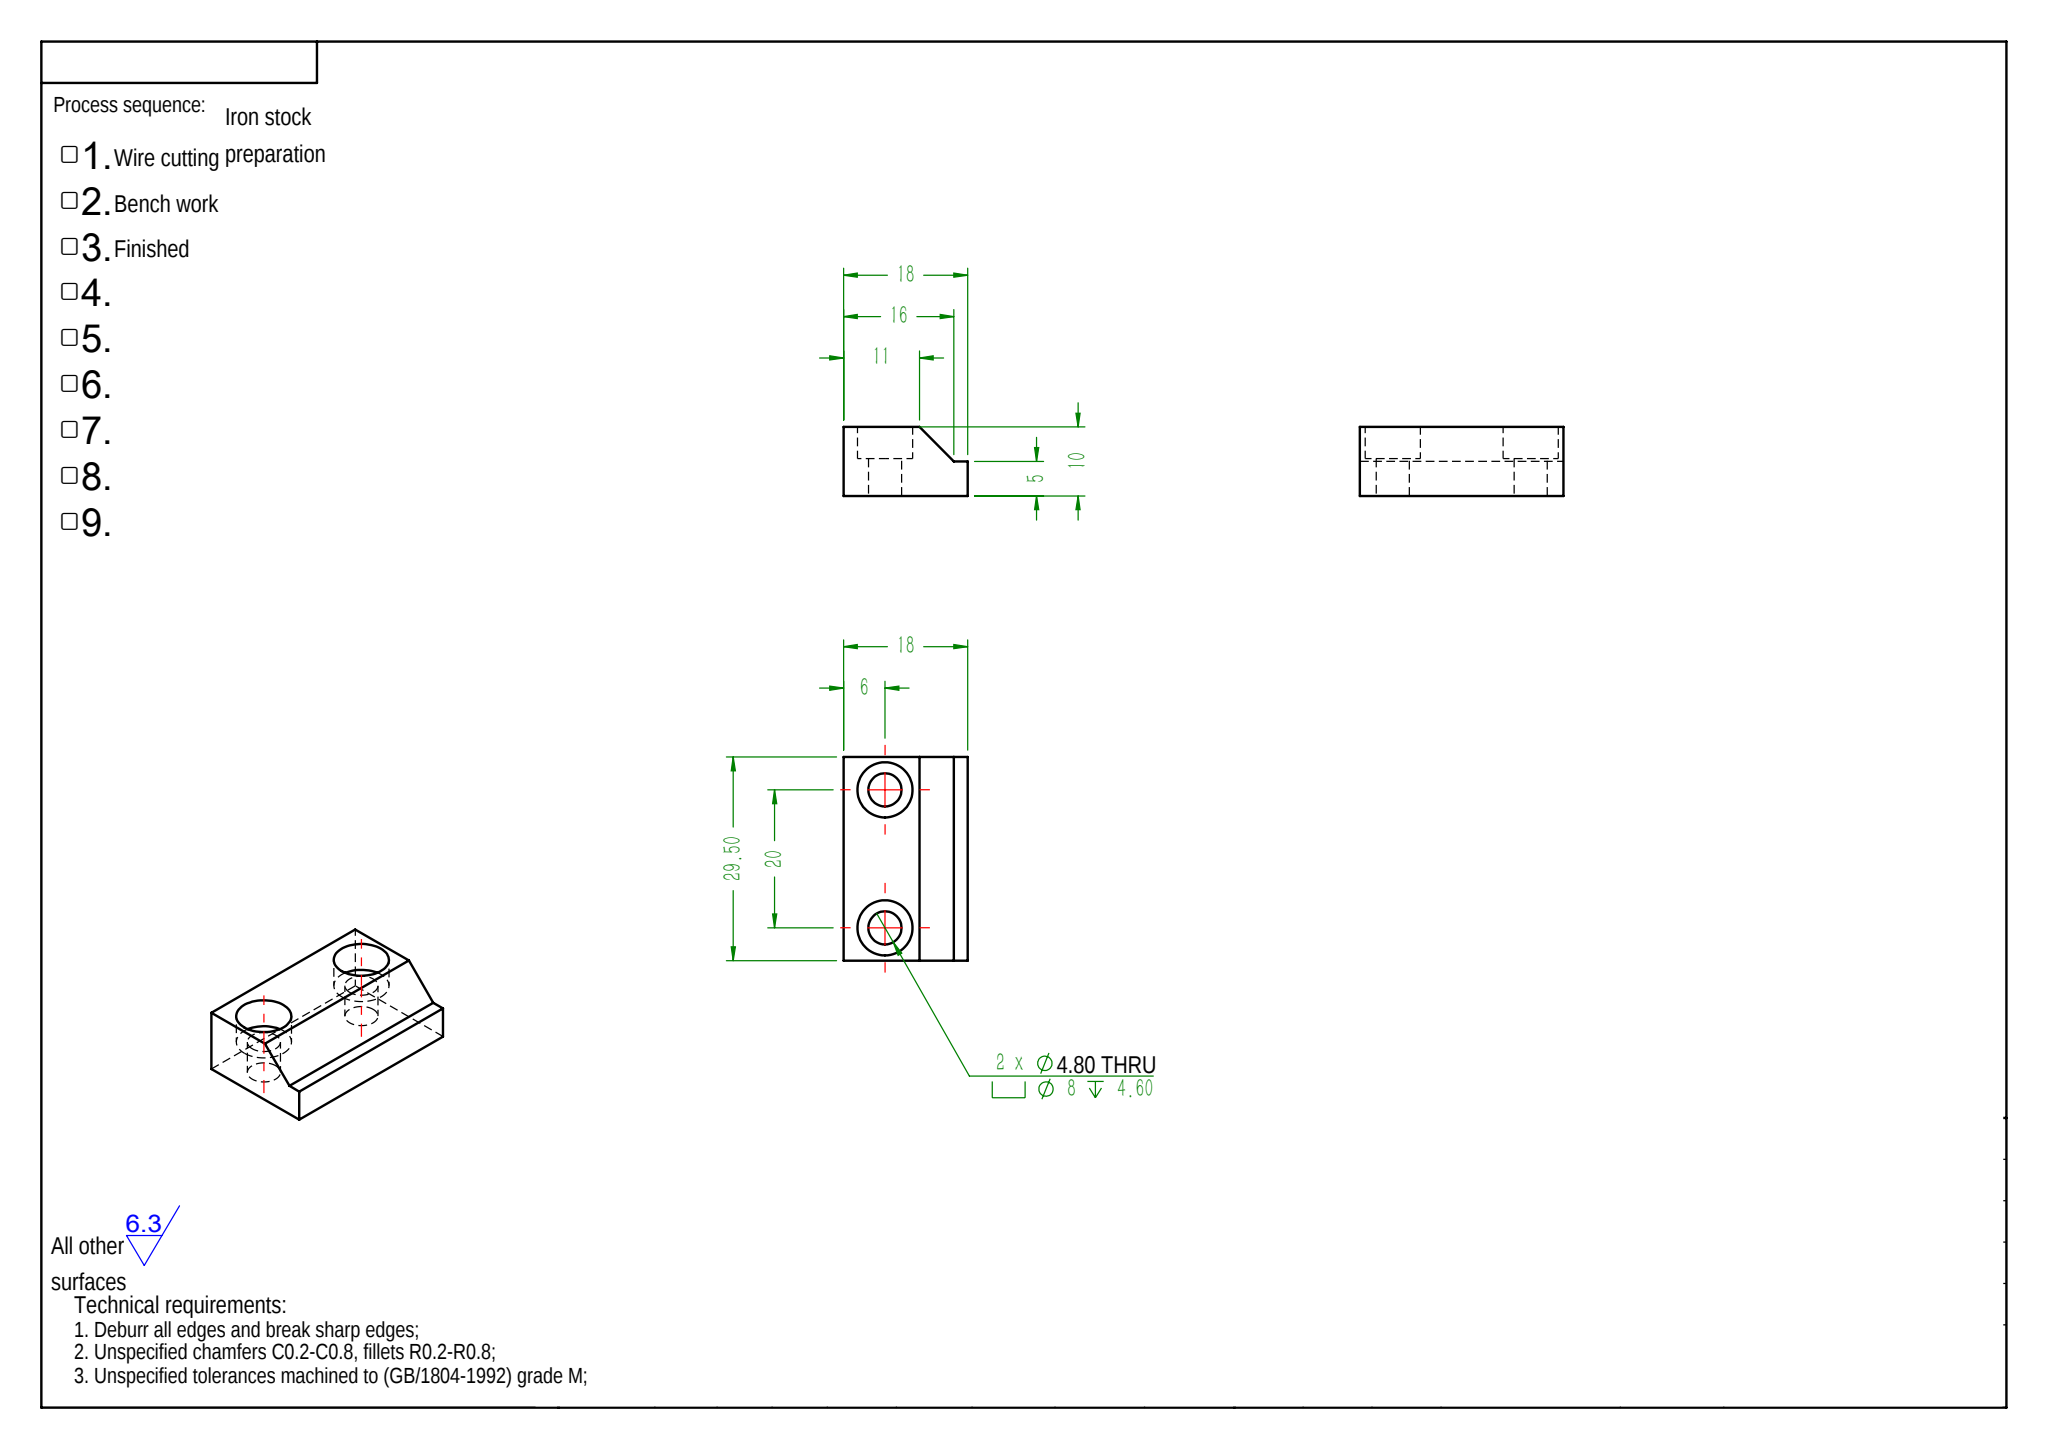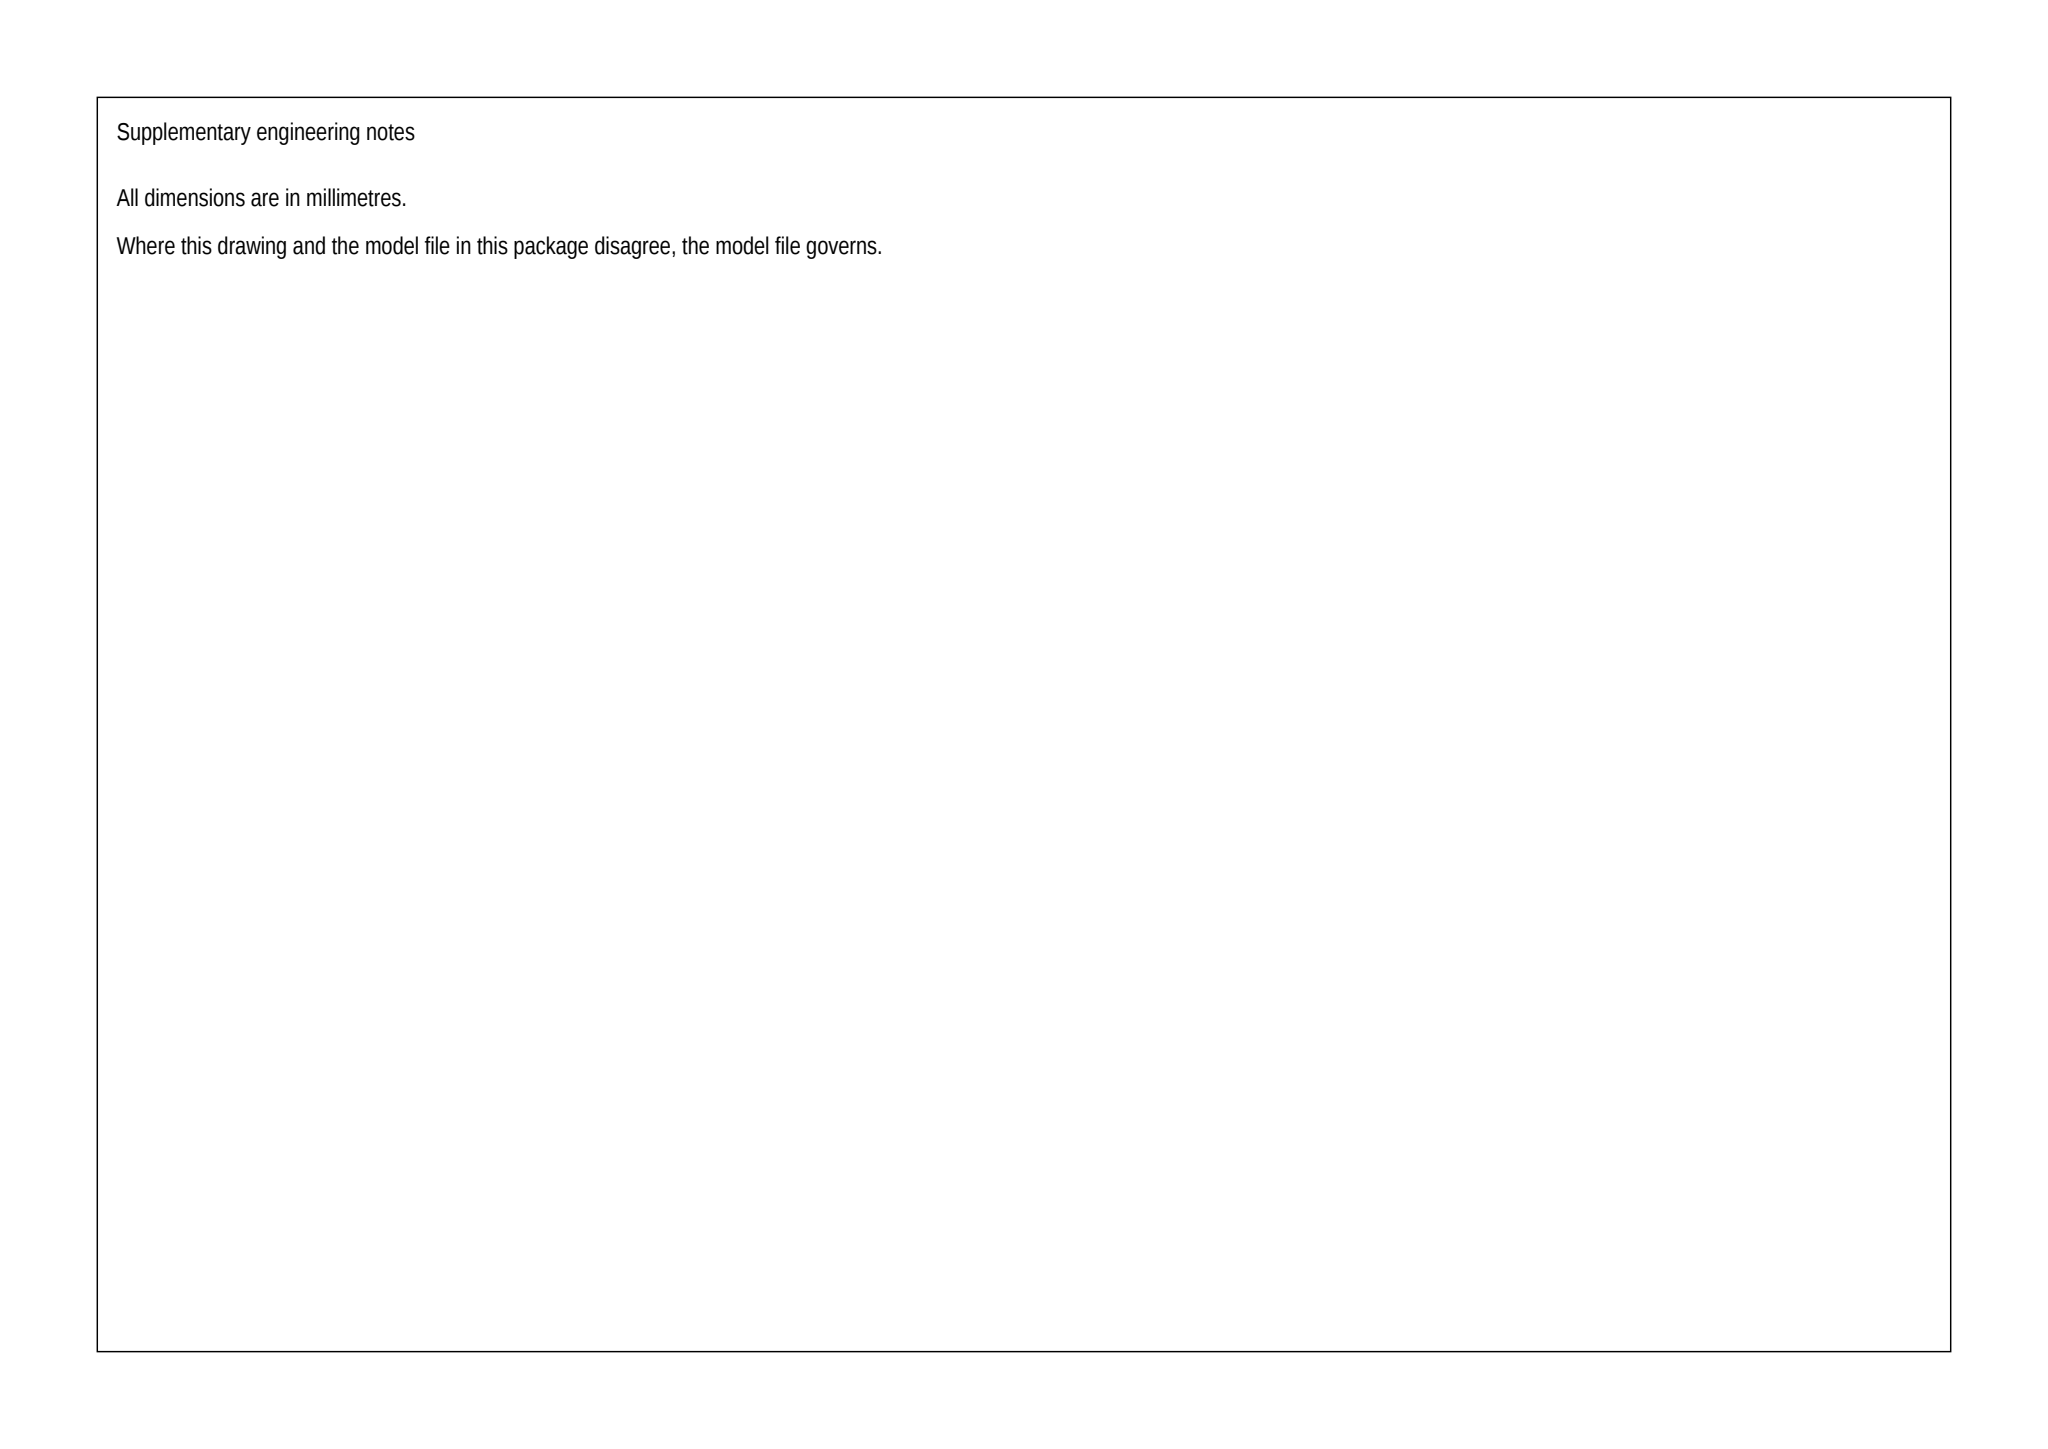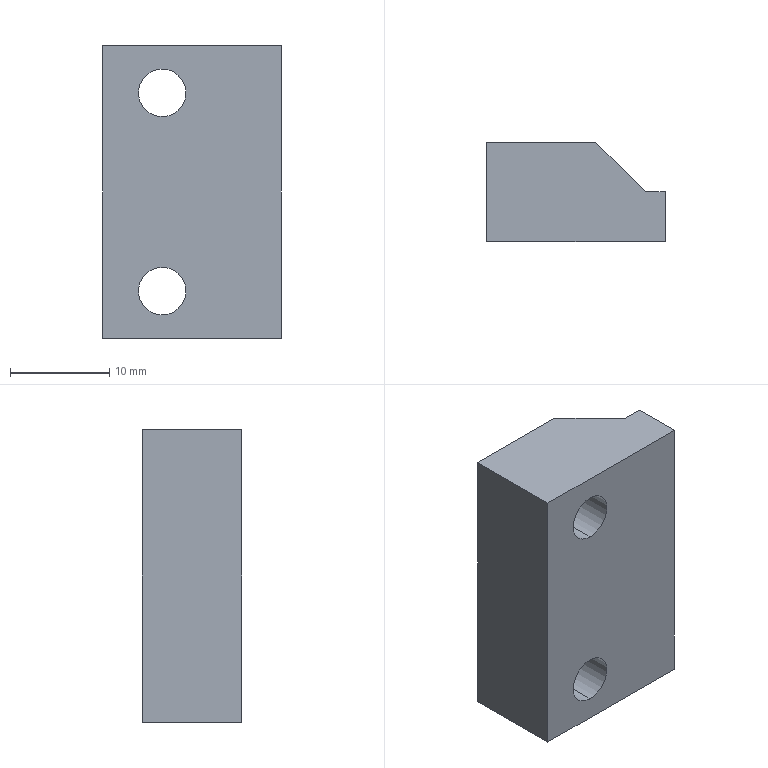Part | SolidWorks | mm | 1 solid | 18 faces | box 18 x 10 x 29.5 mm | volume 3988 mm3 | plane 10 | cylinder 8 | commonest cylinder face diameters 8 x4 4.8 x4
build123d program:
from build123d import *

# Parameters (mm, degrees)
SKETCH2_W                                         = 18
SKETCH2_H                                         = 29.5
BOSS_EXTRUDE1_DEPTH                               = 10
CUT_EXTRUDE1_DEPTH                                = 33.423
HOLE_SIZE_ACCORDING_TO_TYPE_1_OF_HEXA_D           = 4.8
HOLE_SIZE_ACCORDING_TO_TYPE_1_OF_HEXA_CBORE_D     = 8
HOLE_SIZE_ACCORDING_TO_TYPE_1_OF_HEXA_CBORE_DEPTH = 4.6


with BuildPart() as part:
    # Sketch2 → Boss-Extrude1 (new body)
    with BuildSketch(Plane(origin=(0, 0, 0), x_dir=(1, 0, 0), z_dir=(0, 1, 0))):
        Rectangle(SKETCH2_W, SKETCH2_H)
    extrude(amount=BOSS_EXTRUDE1_DEPTH)

    # Sketch3 → Cut-Extrude1 (cut, through all)
    with BuildSketch(Plane.XY.offset(14.75)):
        Polygon((9, 5), (7, 5), (2, 10), (9, 10), align=None)
    extrude(amount=-CUT_EXTRUDE1_DEPTH, mode=Mode.SUBTRACT)

    # Hole Size _ according to_ Type 1 of Hexa (through all)
    with Locations(Plane(origin=(0, 10, 0), x_dir=(1, 0, 0), z_dir=(0, 1, 0))):
        with Locations((-3, 10), (-3, -10)):
            CounterBoreHole(HOLE_SIZE_ACCORDING_TO_TYPE_1_OF_HEXA_D / 2, HOLE_SIZE_ACCORDING_TO_TYPE_1_OF_HEXA_CBORE_D / 2, HOLE_SIZE_ACCORDING_TO_TYPE_1_OF_HEXA_CBORE_DEPTH)


solid = part.part
STEP:
#1=CARTESIAN_POINT('',(-3.,5.4,-14.));
#2=VERTEX_POINT('',#1);
#3=CARTESIAN_POINT('',(-3.,5.4,-6.));
#4=VERTEX_POINT('',#3);
#5=CARTESIAN_POINT('',(-3.,5.4,-10.));
#6=DIRECTION('',(0.,1.,0.));
#7=DIRECTION('',(0.,0.,1.));
#8=AXIS2_PLACEMENT_3D('',#5,#6,#7);
#9=CIRCLE('',#8,4.);
#10=EDGE_CURVE('',#2,#4,#9,.T.);
#11=ORIENTED_EDGE('',*,*,#10,.F.);
#12=CARTESIAN_POINT('',(-3.,10.,-14.));
#13=VERTEX_POINT('',#12);
#14=CARTESIAN_POINT('',(-3.,10.,-14.));
#15=DIRECTION('',(0.,1.,0.));
#16=VECTOR('',#15,1000.);
#17=LINE('',#14,#16);
#18=EDGE_CURVE('',#2,#13,#17,.T.);
#19=ORIENTED_EDGE('',*,*,#18,.T.);
#20=CARTESIAN_POINT('',(-3.,10.,-6.));
#21=VERTEX_POINT('',#20);
#22=CARTESIAN_POINT('',(-3.,10.,-10.));
#23=DIRECTION('',(0.,1.,0.));
#24=DIRECTION('',(0.,0.,1.));
#25=AXIS2_PLACEMENT_3D('',#22,#23,#24);
#26=CIRCLE('',#25,4.);
#27=EDGE_CURVE('',#13,#21,#26,.T.);
#28=ORIENTED_EDGE('',*,*,#27,.T.);
#29=CARTESIAN_POINT('',(-3.,10.,-6.));
#30=DIRECTION('',(0.,1.,0.));
#31=VECTOR('',#30,1000.);
#32=LINE('',#29,#31);
#33=EDGE_CURVE('',#4,#21,#32,.T.);
#34=ORIENTED_EDGE('',*,*,#33,.F.);
#35=EDGE_LOOP('',(#11,#19,#28,#34));
#36=FACE_OUTER_BOUND('',#35,.T.);
#37=CARTESIAN_POINT('',(-3.,10.,-10.));
#38=DIRECTION('',(0.,1.,0.));
#39=DIRECTION('',(0.,0.,1.));
#40=AXIS2_PLACEMENT_3D('',#37,#38,#39);
#41=CYLINDRICAL_SURFACE('',#40,4.);
#42=ADVANCED_FACE('',(#36),#41,.F.);
#43=CARTESIAN_POINT('',(-3.,0.,-7.6));
#44=VERTEX_POINT('',#43);
#45=CARTESIAN_POINT('',(-3.,0.,-12.4));
#46=VERTEX_POINT('',#45);
#47=CARTESIAN_POINT('',(-3.,0.,-10.));
#48=DIRECTION('',(0.,-1.,0.));
#49=DIRECTION('',(0.,0.,-1.));
#50=AXIS2_PLACEMENT_3D('',#47,#48,#49);
#51=CIRCLE('',#50,2.4);
#52=EDGE_CURVE('',#44,#46,#51,.T.);
#53=ORIENTED_EDGE('',*,*,#52,.T.);
#54=CARTESIAN_POINT('',(-3.,5.4,-12.4));
#55=VERTEX_POINT('',#54);
#56=CARTESIAN_POINT('',(-3.,10.,-12.4));
#57=DIRECTION('',(0.,1.,0.));
#58=VECTOR('',#57,1000.);
#59=LINE('',#56,#58);
#60=EDGE_CURVE('',#46,#55,#59,.T.);
#61=ORIENTED_EDGE('',*,*,#60,.T.);
#62=CARTESIAN_POINT('',(-3.,5.4,-7.6));
#63=VERTEX_POINT('',#62);
#64=CARTESIAN_POINT('',(-3.,5.4,-10.));
#65=DIRECTION('',(0.,1.,0.));
#66=DIRECTION('',(0.,0.,1.));
#67=AXIS2_PLACEMENT_3D('',#64,#65,#66);
#68=CIRCLE('',#67,2.4);
#69=EDGE_CURVE('',#55,#63,#68,.T.);
#70=ORIENTED_EDGE('',*,*,#69,.T.);
#71=CARTESIAN_POINT('',(-3.,10.,-7.6));
#72=DIRECTION('',(0.,1.,0.));
#73=VECTOR('',#72,1000.);
#74=LINE('',#71,#73);
#75=EDGE_CURVE('',#44,#63,#74,.T.);
#76=ORIENTED_EDGE('',*,*,#75,.F.);
#77=EDGE_LOOP('',(#53,#61,#70,#76));
#78=FACE_OUTER_BOUND('',#77,.T.);
#79=CARTESIAN_POINT('',(-3.,10.,-10.));
#80=DIRECTION('',(0.,1.,0.));
#81=DIRECTION('',(0.,0.,1.));
#82=AXIS2_PLACEMENT_3D('',#79,#80,#81);
#83=CYLINDRICAL_SURFACE('',#82,2.4);
#84=ADVANCED_FACE('',(#78),#83,.F.);
#85=CARTESIAN_POINT('',(-3.,5.4,6.));
#86=VERTEX_POINT('',#85);
#87=CARTESIAN_POINT('',(-3.,5.4,14.));
#88=VERTEX_POINT('',#87);
#89=CARTESIAN_POINT('',(-3.,5.4,10.));
#90=DIRECTION('',(0.,1.,0.));
#91=DIRECTION('',(0.,0.,1.));
#92=AXIS2_PLACEMENT_3D('',#89,#90,#91);
#93=CIRCLE('',#92,4.);
#94=EDGE_CURVE('',#86,#88,#93,.T.);
#95=ORIENTED_EDGE('',*,*,#94,.F.);
#96=CARTESIAN_POINT('',(-3.,10.,6.));
#97=VERTEX_POINT('',#96);
#98=CARTESIAN_POINT('',(-3.,10.,6.));
#99=DIRECTION('',(0.,1.,0.));
#100=VECTOR('',#99,1000.);
#101=LINE('',#98,#100);
#102=EDGE_CURVE('',#86,#97,#101,.T.);
#103=ORIENTED_EDGE('',*,*,#102,.T.);
#104=CARTESIAN_POINT('',(-3.,10.,14.));
#105=VERTEX_POINT('',#104);
#106=CARTESIAN_POINT('',(-3.,10.,10.));
#107=DIRECTION('',(0.,1.,0.));
#108=DIRECTION('',(0.,0.,1.));
#109=AXIS2_PLACEMENT_3D('',#106,#107,#108);
#110=CIRCLE('',#109,4.);
#111=EDGE_CURVE('',#97,#105,#110,.T.);
#112=ORIENTED_EDGE('',*,*,#111,.T.);
#113=CARTESIAN_POINT('',(-3.,10.,14.));
#114=DIRECTION('',(0.,1.,0.));
#115=VECTOR('',#114,1000.);
#116=LINE('',#113,#115);
#117=EDGE_CURVE('',#88,#105,#116,.T.);
#118=ORIENTED_EDGE('',*,*,#117,.F.);
#119=EDGE_LOOP('',(#95,#103,#112,#118));
#120=FACE_OUTER_BOUND('',#119,.T.);
#121=CARTESIAN_POINT('',(-3.,10.,10.));
#122=DIRECTION('',(0.,1.,0.));
#123=DIRECTION('',(0.,0.,1.));
#124=AXIS2_PLACEMENT_3D('',#121,#122,#123);
#125=CYLINDRICAL_SURFACE('',#124,4.);
#126=ADVANCED_FACE('',(#120),#125,.F.);
#127=CARTESIAN_POINT('',(-3.,0.,12.4));
#128=VERTEX_POINT('',#127);
#129=CARTESIAN_POINT('',(-3.,0.,7.6));
#130=VERTEX_POINT('',#129);
#131=CARTESIAN_POINT('',(-3.,0.,10.));
#132=DIRECTION('',(0.,-1.,0.));
#133=DIRECTION('',(0.,0.,-1.));
#134=AXIS2_PLACEMENT_3D('',#131,#132,#133);
#135=CIRCLE('',#134,2.4);
#136=EDGE_CURVE('',#128,#130,#135,.T.);
#137=ORIENTED_EDGE('',*,*,#136,.T.);
#138=CARTESIAN_POINT('',(-3.,5.4,7.6));
#139=VERTEX_POINT('',#138);
#140=CARTESIAN_POINT('',(-3.,10.,7.6));
#141=DIRECTION('',(0.,1.,0.));
#142=VECTOR('',#141,1000.);
#143=LINE('',#140,#142);
#144=EDGE_CURVE('',#130,#139,#143,.T.);
#145=ORIENTED_EDGE('',*,*,#144,.T.);
#146=CARTESIAN_POINT('',(-3.,5.4,12.4));
#147=VERTEX_POINT('',#146);
#148=CARTESIAN_POINT('',(-3.,5.4,10.));
#149=DIRECTION('',(0.,1.,0.));
#150=DIRECTION('',(0.,0.,1.));
#151=AXIS2_PLACEMENT_3D('',#148,#149,#150);
#152=CIRCLE('',#151,2.4);
#153=EDGE_CURVE('',#139,#147,#152,.T.);
#154=ORIENTED_EDGE('',*,*,#153,.T.);
#155=CARTESIAN_POINT('',(-3.,10.,12.4));
#156=DIRECTION('',(0.,1.,0.));
#157=VECTOR('',#156,1000.);
#158=LINE('',#155,#157);
#159=EDGE_CURVE('',#128,#147,#158,.T.);
#160=ORIENTED_EDGE('',*,*,#159,.F.);
#161=EDGE_LOOP('',(#137,#145,#154,#160));
#162=FACE_OUTER_BOUND('',#161,.T.);
#163=CARTESIAN_POINT('',(-3.,10.,10.));
#164=DIRECTION('',(0.,1.,0.));
#165=DIRECTION('',(0.,0.,1.));
#166=AXIS2_PLACEMENT_3D('',#163,#164,#165);
#167=CYLINDRICAL_SURFACE('',#166,2.4);
#168=ADVANCED_FACE('',(#162),#167,.F.);
#169=CARTESIAN_POINT('',(-9.,0.,-14.75));
#170=VERTEX_POINT('',#169);
#171=CARTESIAN_POINT('',(-9.,0.,14.75));
#172=VERTEX_POINT('',#171);
#173=CARTESIAN_POINT('',(-9.,0.,-14.75));
#174=DIRECTION('',(0.,0.,1.));
#175=VECTOR('',#174,1000.);
#176=LINE('',#173,#175);
#177=EDGE_CURVE('',#170,#172,#176,.T.);
#178=ORIENTED_EDGE('',*,*,#177,.T.);
#179=CARTESIAN_POINT('',(-9.,10.,14.75));
#180=VERTEX_POINT('',#179);
#181=CARTESIAN_POINT('',(-9.,10.,14.75));
#182=DIRECTION('',(0.,-1.,0.));
#183=VECTOR('',#182,1000.);
#184=LINE('',#181,#183);
#185=EDGE_CURVE('',#180,#172,#184,.T.);
#186=ORIENTED_EDGE('',*,*,#185,.F.);
#187=CARTESIAN_POINT('',(-9.,10.,-14.75));
#188=VERTEX_POINT('',#187);
#189=CARTESIAN_POINT('',(-9.,10.,-14.75));
#190=DIRECTION('',(0.,0.,1.));
#191=VECTOR('',#190,1000.);
#192=LINE('',#189,#191);
#193=EDGE_CURVE('',#188,#180,#192,.T.);
#194=ORIENTED_EDGE('',*,*,#193,.F.);
#195=CARTESIAN_POINT('',(-9.,10.,-14.75));
#196=DIRECTION('',(0.,-1.,0.));
#197=VECTOR('',#196,1000.);
#198=LINE('',#195,#197);
#199=EDGE_CURVE('',#188,#170,#198,.T.);
#200=ORIENTED_EDGE('',*,*,#199,.T.);
#201=EDGE_LOOP('',(#178,#186,#194,#200));
#202=FACE_OUTER_BOUND('',#201,.T.);
#203=CARTESIAN_POINT('',(-9.,10.,-14.75));
#204=DIRECTION('',(1.,0.,0.));
#205=DIRECTION('',(0.,0.,-1.));
#206=AXIS2_PLACEMENT_3D('',#203,#204,#205);
#207=PLANE('',#206);
#208=ADVANCED_FACE('',(#202),#207,.F.);
#209=CARTESIAN_POINT('',(9.,5.,14.75));
#210=VERTEX_POINT('',#209);
#211=CARTESIAN_POINT('',(9.,0.,14.75));
#212=VERTEX_POINT('',#211);
#213=CARTESIAN_POINT('',(9.,10.,14.75));
#214=DIRECTION('',(0.,-1.,0.));
#215=VECTOR('',#214,1000.);
#216=LINE('',#213,#215);
#217=EDGE_CURVE('',#210,#212,#216,.T.);
#218=ORIENTED_EDGE('',*,*,#217,.F.);
#219=CARTESIAN_POINT('',(7.,5.,14.75));
#220=VERTEX_POINT('',#219);
#221=CARTESIAN_POINT('',(9.,5.,14.75));
#222=DIRECTION('',(1.,0.,0.));
#223=VECTOR('',#222,1000.);
#224=LINE('',#221,#223);
#225=EDGE_CURVE('',#220,#210,#224,.T.);
#226=ORIENTED_EDGE('',*,*,#225,.F.);
#227=CARTESIAN_POINT('',(2.,10.,14.75));
#228=VERTEX_POINT('',#227);
#229=CARTESIAN_POINT('',(7.,5.,14.75));
#230=DIRECTION('',(0.7071,-0.7071,0.));
#231=VECTOR('',#230,1000.);
#232=LINE('',#229,#231);
#233=EDGE_CURVE('',#228,#220,#232,.T.);
#234=ORIENTED_EDGE('',*,*,#233,.F.);
#235=CARTESIAN_POINT('',(9.,10.,14.75));
#236=DIRECTION('',(1.,0.,0.));
#237=VECTOR('',#236,1000.);
#238=LINE('',#235,#237);
#239=EDGE_CURVE('',#180,#228,#238,.T.);
#240=ORIENTED_EDGE('',*,*,#239,.F.);
#241=ORIENTED_EDGE('',*,*,#185,.T.);
#242=CARTESIAN_POINT('',(9.,0.,14.75));
#243=DIRECTION('',(1.,0.,0.));
#244=VECTOR('',#243,1000.);
#245=LINE('',#242,#244);
#246=EDGE_CURVE('',#172,#212,#245,.T.);
#247=ORIENTED_EDGE('',*,*,#246,.T.);
#248=EDGE_LOOP('',(#218,#226,#234,#240,#241,#247));
#249=FACE_OUTER_BOUND('',#248,.T.);
#250=CARTESIAN_POINT('',(9.,10.,14.75));
#251=DIRECTION('',(0.,0.,-1.));
#252=DIRECTION('',(-1.,0.,0.));
#253=AXIS2_PLACEMENT_3D('',#250,#251,#252);
#254=PLANE('',#253);
#255=ADVANCED_FACE('',(#249),#254,.F.);
#256=CARTESIAN_POINT('',(9.,5.,-14.75));
#257=VERTEX_POINT('',#256);
#258=CARTESIAN_POINT('',(9.,0.,-14.75));
#259=VERTEX_POINT('',#258);
#260=CARTESIAN_POINT('',(9.,10.,-14.75));
#261=DIRECTION('',(0.,-1.,0.));
#262=VECTOR('',#261,1000.);
#263=LINE('',#260,#262);
#264=EDGE_CURVE('',#257,#259,#263,.T.);
#265=ORIENTED_EDGE('',*,*,#264,.F.);
#266=CARTESIAN_POINT('',(9.,5.,-14.75));
#267=DIRECTION('',(0.,0.,1.));
#268=VECTOR('',#267,1000.);
#269=LINE('',#266,#268);
#270=EDGE_CURVE('',#257,#210,#269,.T.);
#271=ORIENTED_EDGE('',*,*,#270,.T.);
#272=ORIENTED_EDGE('',*,*,#217,.T.);
#273=CARTESIAN_POINT('',(9.,0.,-14.75));
#274=DIRECTION('',(0.,0.,-1.));
#275=VECTOR('',#274,1000.);
#276=LINE('',#273,#275);
#277=EDGE_CURVE('',#212,#259,#276,.T.);
#278=ORIENTED_EDGE('',*,*,#277,.T.);
#279=EDGE_LOOP('',(#265,#271,#272,#278));
#280=FACE_OUTER_BOUND('',#279,.T.);
#281=CARTESIAN_POINT('',(9.,10.,-14.75));
#282=DIRECTION('',(-1.,0.,0.));
#283=DIRECTION('',(0.,0.,1.));
#284=AXIS2_PLACEMENT_3D('',#281,#282,#283);
#285=PLANE('',#284);
#286=ADVANCED_FACE('',(#280),#285,.F.);
#287=CARTESIAN_POINT('',(2.,10.,-14.75));
#288=VERTEX_POINT('',#287);
#289=CARTESIAN_POINT('',(7.,5.,-14.75));
#290=VERTEX_POINT('',#289);
#291=CARTESIAN_POINT('',(7.,5.,-14.75));
#292=DIRECTION('',(0.7071,-0.7071,0.));
#293=VECTOR('',#292,1000.);
#294=LINE('',#291,#293);
#295=EDGE_CURVE('',#288,#290,#294,.T.);
#296=ORIENTED_EDGE('',*,*,#295,.T.);
#297=CARTESIAN_POINT('',(9.,5.,-14.75));
#298=DIRECTION('',(1.,0.,0.));
#299=VECTOR('',#298,1000.);
#300=LINE('',#297,#299);
#301=EDGE_CURVE('',#290,#257,#300,.T.);
#302=ORIENTED_EDGE('',*,*,#301,.T.);
#303=ORIENTED_EDGE('',*,*,#264,.T.);
#304=CARTESIAN_POINT('',(9.,0.,-14.75));
#305=DIRECTION('',(-1.,0.,0.));
#306=VECTOR('',#305,1000.);
#307=LINE('',#304,#306);
#308=EDGE_CURVE('',#259,#170,#307,.T.);
#309=ORIENTED_EDGE('',*,*,#308,.T.);
#310=ORIENTED_EDGE('',*,*,#199,.F.);
#311=CARTESIAN_POINT('',(9.,10.,-14.75));
#312=DIRECTION('',(-1.,0.,0.));
#313=VECTOR('',#312,1000.);
#314=LINE('',#311,#313);
#315=EDGE_CURVE('',#288,#188,#314,.T.);
#316=ORIENTED_EDGE('',*,*,#315,.F.);
#317=EDGE_LOOP('',(#296,#302,#303,#309,#310,#316));
#318=FACE_OUTER_BOUND('',#317,.T.);
#319=CARTESIAN_POINT('',(9.,10.,-14.75));
#320=DIRECTION('',(0.,0.,1.));
#321=DIRECTION('',(1.,0.,0.));
#322=AXIS2_PLACEMENT_3D('',#319,#320,#321);
#323=PLANE('',#322);
#324=ADVANCED_FACE('',(#318),#323,.F.);
#325=CARTESIAN_POINT('',(-3.,10.,-10.));
#326=DIRECTION('',(0.,1.,0.));
#327=DIRECTION('',(0.,0.,1.));
#328=AXIS2_PLACEMENT_3D('',#325,#326,#327);
#329=CIRCLE('',#328,4.);
#330=EDGE_CURVE('',#21,#13,#329,.T.);
#331=ORIENTED_EDGE('',*,*,#330,.F.);
#332=ORIENTED_EDGE('',*,*,#27,.F.);
#333=EDGE_LOOP('',(#331,#332));
#334=FACE_BOUND('',#333,.T.);
#335=CARTESIAN_POINT('',(-3.,10.,10.));
#336=DIRECTION('',(0.,1.,0.));
#337=DIRECTION('',(0.,0.,1.));
#338=AXIS2_PLACEMENT_3D('',#335,#336,#337);
#339=CIRCLE('',#338,4.);
#340=EDGE_CURVE('',#105,#97,#339,.T.);
#341=ORIENTED_EDGE('',*,*,#340,.F.);
#342=ORIENTED_EDGE('',*,*,#111,.F.);
#343=EDGE_LOOP('',(#341,#342));
#344=FACE_BOUND('',#343,.T.);
#345=ORIENTED_EDGE('',*,*,#239,.T.);
#346=CARTESIAN_POINT('',(2.,10.,-14.75));
#347=DIRECTION('',(0.,0.,1.));
#348=VECTOR('',#347,1000.);
#349=LINE('',#346,#348);
#350=EDGE_CURVE('',#288,#228,#349,.T.);
#351=ORIENTED_EDGE('',*,*,#350,.F.);
#352=ORIENTED_EDGE('',*,*,#315,.T.);
#353=ORIENTED_EDGE('',*,*,#193,.T.);
#354=EDGE_LOOP('',(#345,#351,#352,#353));
#355=FACE_OUTER_BOUND('',#354,.T.);
#356=CARTESIAN_POINT('',(0.,10.,0.));
#357=DIRECTION('',(0.,-1.,0.));
#358=DIRECTION('',(0.,0.,-1.));
#359=AXIS2_PLACEMENT_3D('',#356,#357,#358);
#360=PLANE('',#359);
#361=ADVANCED_FACE('',(#334,#344,#355),#360,.F.);
#362=ORIENTED_EDGE('',*,*,#52,.F.);
#363=CARTESIAN_POINT('',(-3.,0.,-10.));
#364=DIRECTION('',(0.,-1.,0.));
#365=DIRECTION('',(0.,0.,-1.));
#366=AXIS2_PLACEMENT_3D('',#363,#364,#365);
#367=CIRCLE('',#366,2.4);
#368=EDGE_CURVE('',#46,#44,#367,.T.);
#369=ORIENTED_EDGE('',*,*,#368,.F.);
#370=EDGE_LOOP('',(#362,#369));
#371=FACE_BOUND('',#370,.T.);
#372=ORIENTED_EDGE('',*,*,#136,.F.);
#373=CARTESIAN_POINT('',(-3.,0.,10.));
#374=DIRECTION('',(0.,-1.,0.));
#375=DIRECTION('',(0.,0.,-1.));
#376=AXIS2_PLACEMENT_3D('',#373,#374,#375);
#377=CIRCLE('',#376,2.4);
#378=EDGE_CURVE('',#130,#128,#377,.T.);
#379=ORIENTED_EDGE('',*,*,#378,.F.);
#380=EDGE_LOOP('',(#372,#379));
#381=FACE_BOUND('',#380,.T.);
#382=ORIENTED_EDGE('',*,*,#177,.F.);
#383=ORIENTED_EDGE('',*,*,#308,.F.);
#384=ORIENTED_EDGE('',*,*,#277,.F.);
#385=ORIENTED_EDGE('',*,*,#246,.F.);
#386=EDGE_LOOP('',(#382,#383,#384,#385));
#387=FACE_OUTER_BOUND('',#386,.T.);
#388=CARTESIAN_POINT('',(0.,0.,0.));
#389=DIRECTION('',(0.,-1.,0.));
#390=DIRECTION('',(0.,0.,-1.));
#391=AXIS2_PLACEMENT_3D('',#388,#389,#390);
#392=PLANE('',#391);
#393=ADVANCED_FACE('',(#371,#381,#387),#392,.T.);
#394=ORIENTED_EDGE('',*,*,#225,.T.);
#395=ORIENTED_EDGE('',*,*,#270,.F.);
#396=ORIENTED_EDGE('',*,*,#301,.F.);
#397=CARTESIAN_POINT('',(7.,5.,-14.75));
#398=DIRECTION('',(0.,0.,1.));
#399=VECTOR('',#398,1000.);
#400=LINE('',#397,#399);
#401=EDGE_CURVE('',#290,#220,#400,.T.);
#402=ORIENTED_EDGE('',*,*,#401,.T.);
#403=EDGE_LOOP('',(#394,#395,#396,#402));
#404=FACE_OUTER_BOUND('',#403,.T.);
#405=CARTESIAN_POINT('',(9.,5.,-14.75));
#406=DIRECTION('',(0.,-1.,0.));
#407=DIRECTION('',(1.,0.,0.));
#408=AXIS2_PLACEMENT_3D('',#405,#406,#407);
#409=PLANE('',#408);
#410=ADVANCED_FACE('',(#404),#409,.F.);
#411=ORIENTED_EDGE('',*,*,#233,.T.);
#412=ORIENTED_EDGE('',*,*,#401,.F.);
#413=ORIENTED_EDGE('',*,*,#295,.F.);
#414=ORIENTED_EDGE('',*,*,#350,.T.);
#415=EDGE_LOOP('',(#411,#412,#413,#414));
#416=FACE_OUTER_BOUND('',#415,.T.);
#417=CARTESIAN_POINT('',(7.,5.,-14.75));
#418=DIRECTION('',(-0.7071,-0.7071,0.));
#419=DIRECTION('',(0.7071,-0.7071,0.));
#420=AXIS2_PLACEMENT_3D('',#417,#418,#419);
#421=PLANE('',#420);
#422=ADVANCED_FACE('',(#416),#421,.F.);
#423=ORIENTED_EDGE('',*,*,#144,.F.);
#424=ORIENTED_EDGE('',*,*,#378,.T.);
#425=ORIENTED_EDGE('',*,*,#159,.T.);
#426=CARTESIAN_POINT('',(-3.,5.4,10.));
#427=DIRECTION('',(0.,1.,0.));
#428=DIRECTION('',(0.,0.,1.));
#429=AXIS2_PLACEMENT_3D('',#426,#427,#428);
#430=CIRCLE('',#429,2.4);
#431=EDGE_CURVE('',#147,#139,#430,.T.);
#432=ORIENTED_EDGE('',*,*,#431,.T.);
#433=EDGE_LOOP('',(#423,#424,#425,#432));
#434=FACE_OUTER_BOUND('',#433,.T.);
#435=CARTESIAN_POINT('',(-3.,10.,10.));
#436=DIRECTION('',(0.,1.,0.));
#437=DIRECTION('',(0.,0.,1.));
#438=AXIS2_PLACEMENT_3D('',#435,#436,#437);
#439=CYLINDRICAL_SURFACE('',#438,2.4);
#440=ADVANCED_FACE('',(#434),#439,.F.);
#441=ORIENTED_EDGE('',*,*,#431,.F.);
#442=ORIENTED_EDGE('',*,*,#153,.F.);
#443=EDGE_LOOP('',(#441,#442));
#444=FACE_BOUND('',#443,.T.);
#445=CARTESIAN_POINT('',(-3.,5.4,10.));
#446=DIRECTION('',(0.,1.,0.));
#447=DIRECTION('',(0.,0.,1.));
#448=AXIS2_PLACEMENT_3D('',#445,#446,#447);
#449=CIRCLE('',#448,4.);
#450=EDGE_CURVE('',#88,#86,#449,.T.);
#451=ORIENTED_EDGE('',*,*,#450,.T.);
#452=ORIENTED_EDGE('',*,*,#94,.T.);
#453=EDGE_LOOP('',(#451,#452));
#454=FACE_OUTER_BOUND('',#453,.T.);
#455=CARTESIAN_POINT('',(-0.6,5.4,10.));
#456=DIRECTION('',(0.,-1.,0.));
#457=DIRECTION('',(0.,0.,-1.));
#458=AXIS2_PLACEMENT_3D('',#455,#456,#457);
#459=PLANE('',#458);
#460=ADVANCED_FACE('',(#444,#454),#459,.F.);
#461=ORIENTED_EDGE('',*,*,#102,.F.);
#462=ORIENTED_EDGE('',*,*,#450,.F.);
#463=ORIENTED_EDGE('',*,*,#117,.T.);
#464=ORIENTED_EDGE('',*,*,#340,.T.);
#465=EDGE_LOOP('',(#461,#462,#463,#464));
#466=FACE_OUTER_BOUND('',#465,.T.);
#467=CARTESIAN_POINT('',(-3.,10.,10.));
#468=DIRECTION('',(0.,1.,0.));
#469=DIRECTION('',(0.,0.,1.));
#470=AXIS2_PLACEMENT_3D('',#467,#468,#469);
#471=CYLINDRICAL_SURFACE('',#470,4.);
#472=ADVANCED_FACE('',(#466),#471,.F.);
#473=ORIENTED_EDGE('',*,*,#60,.F.);
#474=ORIENTED_EDGE('',*,*,#368,.T.);
#475=ORIENTED_EDGE('',*,*,#75,.T.);
#476=CARTESIAN_POINT('',(-3.,5.4,-10.));
#477=DIRECTION('',(0.,1.,0.));
#478=DIRECTION('',(0.,0.,1.));
#479=AXIS2_PLACEMENT_3D('',#476,#477,#478);
#480=CIRCLE('',#479,2.4);
#481=EDGE_CURVE('',#63,#55,#480,.T.);
#482=ORIENTED_EDGE('',*,*,#481,.T.);
#483=EDGE_LOOP('',(#473,#474,#475,#482));
#484=FACE_OUTER_BOUND('',#483,.T.);
#485=CARTESIAN_POINT('',(-3.,10.,-10.));
#486=DIRECTION('',(0.,1.,0.));
#487=DIRECTION('',(0.,0.,1.));
#488=AXIS2_PLACEMENT_3D('',#485,#486,#487);
#489=CYLINDRICAL_SURFACE('',#488,2.4);
#490=ADVANCED_FACE('',(#484),#489,.F.);
#491=ORIENTED_EDGE('',*,*,#481,.F.);
#492=ORIENTED_EDGE('',*,*,#69,.F.);
#493=EDGE_LOOP('',(#491,#492));
#494=FACE_BOUND('',#493,.T.);
#495=CARTESIAN_POINT('',(-3.,5.4,-10.));
#496=DIRECTION('',(0.,1.,0.));
#497=DIRECTION('',(0.,0.,1.));
#498=AXIS2_PLACEMENT_3D('',#495,#496,#497);
#499=CIRCLE('',#498,4.);
#500=EDGE_CURVE('',#4,#2,#499,.T.);
#501=ORIENTED_EDGE('',*,*,#500,.T.);
#502=ORIENTED_EDGE('',*,*,#10,.T.);
#503=EDGE_LOOP('',(#501,#502));
#504=FACE_OUTER_BOUND('',#503,.T.);
#505=CARTESIAN_POINT('',(-0.6,5.4,-10.));
#506=DIRECTION('',(0.,-1.,0.));
#507=DIRECTION('',(0.,0.,-1.));
#508=AXIS2_PLACEMENT_3D('',#505,#506,#507);
#509=PLANE('',#508);
#510=ADVANCED_FACE('',(#494,#504),#509,.F.);
#511=ORIENTED_EDGE('',*,*,#18,.F.);
#512=ORIENTED_EDGE('',*,*,#500,.F.);
#513=ORIENTED_EDGE('',*,*,#33,.T.);
#514=ORIENTED_EDGE('',*,*,#330,.T.);
#515=EDGE_LOOP('',(#511,#512,#513,#514));
#516=FACE_OUTER_BOUND('',#515,.T.);
#517=CARTESIAN_POINT('',(-3.,10.,-10.));
#518=DIRECTION('',(0.,1.,0.));
#519=DIRECTION('',(0.,0.,1.));
#520=AXIS2_PLACEMENT_3D('',#517,#518,#519);
#521=CYLINDRICAL_SURFACE('',#520,4.);
#522=ADVANCED_FACE('',(#516),#521,.F.);
#523=CLOSED_SHELL('',(#42,#84,#126,#168,#208,#255,#286,#324,#361,#393,#410,#422,#440,#460,#472,#490,#510,#522));
#524=MANIFOLD_SOLID_BREP('',#523);
#525=CARTESIAN_POINT('',(0.,0.,0.));
#526=DIRECTION('',(0.,0.,1.));
#527=DIRECTION('',(1.,0.,0.));
#528=AXIS2_PLACEMENT_3D('',#525,#526,#527);
#529=(LENGTH_UNIT()NAMED_UNIT(*)SI_UNIT(.MILLI.,.METRE.));
#530=UNCERTAINTY_MEASURE_WITH_UNIT(LENGTH_MEASURE(0.00001),#529,'','');
#531=(NAMED_UNIT(*)PLANE_ANGLE_UNIT()SI_UNIT($,.RADIAN.));
#532=(NAMED_UNIT(*)SI_UNIT($,.STERADIAN.)SOLID_ANGLE_UNIT());
#533=(GEOMETRIC_REPRESENTATION_CONTEXT(3)GLOBAL_UNCERTAINTY_ASSIGNED_CONTEXT((#530))GLOBAL_UNIT_ASSIGNED_CONTEXT((#529,#531,#532))REPRESENTATION_CONTEXT('',''));
#534=ADVANCED_BREP_SHAPE_REPRESENTATION('',(#524,#528),#533);